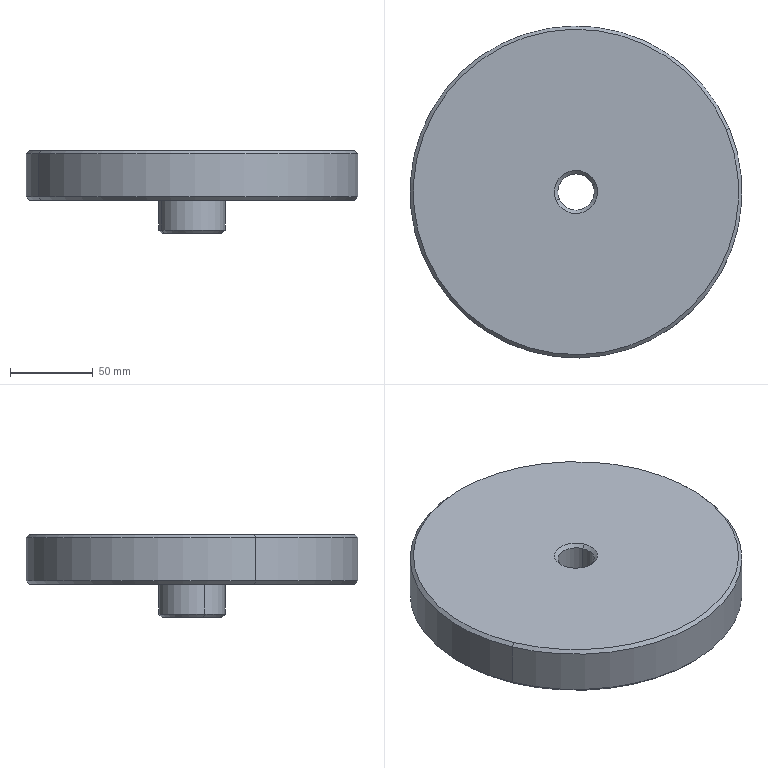Component | SolidWorks | Pinion-1 | 1 solid | 19 faces | box 200 x 200 x 50 mm | volume 945571 mm3 | cone 10 | cylinder 6 | plane 3 | commonest cylinder face diameters 40 x2 200 x2 22 x2 | material 45
build123d program:
from build123d import *

# Parameters (mm, degrees)
CHAMFER1_SIZE = 2


with BuildPart() as part:
    # Sketch1 → Revolve1 (revolve)
    with BuildSketch(Plane.XY, mode=Mode.PRIVATE) as revolve1_sk:
        Polygon((0, 11), (0, 100), (30, 100), (30, 20), (50, 20), (50, 11), align=None)
    revolve(revolve1_sk.sketch.rotate(Axis((0, 0, 0), (1, 0, 0)), 90), axis=Axis((0, 0, 0), (1, 0, 0)))

    # Chamfer1
    chamfer1_edges = [part.edges().sort_by_distance(p)[0] for p in [
        (50, 0, -11),
        (50, 0, -20),
        (30, 0, -100),
        (0, 0, -100),
        (0, 0, -11),
    ]]
    chamfer(chamfer1_edges, length=CHAMFER1_SIZE)


solid = part.part

# Placed as in the assembly
solid = solid.moved(Location((110.202, 126.699, 572.267), (0, 90, 0)))
STEP:
#1=CARTESIAN_POINT('',(7.903,6.466,22.53));
#2=VERTEX_POINT('',#1);
#3=CARTESIAN_POINT('',(0.7747,3.51,22.53));
#4=VERTEX_POINT('',#3);
#5=CARTESIAN_POINT('',(4.339,4.988,22.53));
#6=DIRECTION('',(0.,-0.,1.));
#7=DIRECTION('',(-0.9237,-0.383,0.));
#8=AXIS2_PLACEMENT_3D('',#5,#6,#7);
#9=CIRCLE('',#8,3.858);
#10=EDGE_CURVE('',#2,#4,#9,.T.);
#11=ORIENTED_EDGE('',*,*,#10,.F.);
#12=CARTESIAN_POINT('',(7.975,6.496,22.451));
#13=VERTEX_POINT('',#12);
#14=CARTESIAN_POINT('',(7.903,6.466,22.53));
#15=DIRECTION('',(0.6532,0.2709,-0.7071));
#16=VECTOR('',#15,39.37);
#17=LINE('',#14,#16);
#18=EDGE_CURVE('',#2,#13,#17,.T.);
#19=ORIENTED_EDGE('',*,*,#18,.T.);
#20=CARTESIAN_POINT('',(0.7019,3.48,22.451));
#21=VERTEX_POINT('',#20);
#22=CARTESIAN_POINT('',(4.339,4.988,22.451));
#23=DIRECTION('',(-0.,0.,-1.));
#24=DIRECTION('',(-0.9237,-0.383,0.));
#25=AXIS2_PLACEMENT_3D('',#22,#23,#24);
#26=CIRCLE('',#25,3.937);
#27=EDGE_CURVE('',#21,#13,#26,.T.);
#28=ORIENTED_EDGE('',*,*,#27,.F.);
#29=CARTESIAN_POINT('',(0.7747,3.51,22.53));
#30=DIRECTION('',(-0.6532,-0.2709,-0.7071));
#31=VECTOR('',#30,39.37);
#32=LINE('',#29,#31);
#33=EDGE_CURVE('',#4,#21,#32,.T.);
#34=ORIENTED_EDGE('',*,*,#33,.F.);
#35=EDGE_LOOP('',(#11,#19,#28,#34));
#36=FACE_OUTER_BOUND('',#35,.T.);
#37=CARTESIAN_POINT('',(4.339,4.988,22.53));
#38=DIRECTION('',(-0.,0.,-1.));
#39=DIRECTION('',(-0.9237,-0.383,0.));
#40=AXIS2_PLACEMENT_3D('',#37,#38,#39);
#41=CONICAL_SURFACE('',#40,3.858,0.7854);
#42=ADVANCED_FACE('',(#36),#41,.T.);
#43=CARTESIAN_POINT('',(0.7747,3.51,21.349));
#44=VERTEX_POINT('',#43);
#45=CARTESIAN_POINT('',(7.903,6.466,21.349));
#46=VERTEX_POINT('',#45);
#47=CARTESIAN_POINT('',(4.339,4.988,21.349));
#48=DIRECTION('',(-0.,0.,-1.));
#49=DIRECTION('',(0.9237,0.383,0.));
#50=AXIS2_PLACEMENT_3D('',#47,#48,#49);
#51=CIRCLE('',#50,3.858);
#52=EDGE_CURVE('',#44,#46,#51,.T.);
#53=ORIENTED_EDGE('',*,*,#52,.F.);
#54=CARTESIAN_POINT('',(0.7019,3.48,21.428));
#55=VERTEX_POINT('',#54);
#56=CARTESIAN_POINT('',(0.7019,3.48,21.428));
#57=DIRECTION('',(-0.6532,-0.2709,0.7071));
#58=VECTOR('',#57,39.37);
#59=LINE('',#56,#58);
#60=EDGE_CURVE('',#44,#55,#59,.T.);
#61=ORIENTED_EDGE('',*,*,#60,.T.);
#62=CARTESIAN_POINT('',(7.975,6.496,21.428));
#63=VERTEX_POINT('',#62);
#64=CARTESIAN_POINT('',(4.339,4.988,21.428));
#65=DIRECTION('',(0.,-0.,1.));
#66=DIRECTION('',(0.9237,0.383,0.));
#67=AXIS2_PLACEMENT_3D('',#64,#65,#66);
#68=CIRCLE('',#67,3.937);
#69=EDGE_CURVE('',#63,#55,#68,.T.);
#70=ORIENTED_EDGE('',*,*,#69,.F.);
#71=CARTESIAN_POINT('',(7.975,6.496,21.428));
#72=DIRECTION('',(0.6532,0.2709,0.7071));
#73=VECTOR('',#72,39.37);
#74=LINE('',#71,#73);
#75=EDGE_CURVE('',#46,#63,#74,.T.);
#76=ORIENTED_EDGE('',*,*,#75,.F.);
#77=EDGE_LOOP('',(#53,#61,#70,#76));
#78=FACE_OUTER_BOUND('',#77,.T.);
#79=CARTESIAN_POINT('',(4.339,4.988,21.428));
#80=DIRECTION('',(0.,-0.,1.));
#81=DIRECTION('',(0.9237,0.383,0.));
#82=AXIS2_PLACEMENT_3D('',#79,#80,#81);
#83=CONICAL_SURFACE('',#82,3.937,0.7854);
#84=ADVANCED_FACE('',(#78),#83,.T.);
#85=CARTESIAN_POINT('',(3.684,4.717,20.562));
#86=VERTEX_POINT('',#85);
#87=CARTESIAN_POINT('',(4.993,5.26,20.562));
#88=VERTEX_POINT('',#87);
#89=CARTESIAN_POINT('',(4.339,4.988,20.562));
#90=DIRECTION('',(-0.,0.,-1.));
#91=DIRECTION('',(0.9237,0.383,0.));
#92=AXIS2_PLACEMENT_3D('',#89,#90,#91);
#93=CIRCLE('',#92,0.7087);
#94=EDGE_CURVE('',#86,#88,#93,.T.);
#95=ORIENTED_EDGE('',*,*,#94,.F.);
#96=CARTESIAN_POINT('',(3.611,4.687,20.64));
#97=VERTEX_POINT('',#96);
#98=CARTESIAN_POINT('',(3.611,4.687,20.64));
#99=DIRECTION('',(-0.6532,-0.2709,0.7071));
#100=VECTOR('',#99,39.37);
#101=LINE('',#98,#100);
#102=EDGE_CURVE('',#86,#97,#101,.T.);
#103=ORIENTED_EDGE('',*,*,#102,.T.);
#104=CARTESIAN_POINT('',(5.066,5.29,20.64));
#105=VERTEX_POINT('',#104);
#106=CARTESIAN_POINT('',(4.339,4.988,20.64));
#107=DIRECTION('',(0.,-0.,1.));
#108=DIRECTION('',(0.9237,0.383,0.));
#109=AXIS2_PLACEMENT_3D('',#106,#107,#108);
#110=CIRCLE('',#109,0.7874);
#111=EDGE_CURVE('',#105,#97,#110,.T.);
#112=ORIENTED_EDGE('',*,*,#111,.F.);
#113=CARTESIAN_POINT('',(5.066,5.29,20.64));
#114=DIRECTION('',(0.6532,0.2709,0.7071));
#115=VECTOR('',#114,39.37);
#116=LINE('',#113,#115);
#117=EDGE_CURVE('',#88,#105,#116,.T.);
#118=ORIENTED_EDGE('',*,*,#117,.F.);
#119=EDGE_LOOP('',(#95,#103,#112,#118));
#120=FACE_OUTER_BOUND('',#119,.T.);
#121=CARTESIAN_POINT('',(4.339,4.988,20.64));
#122=DIRECTION('',(0.,-0.,1.));
#123=DIRECTION('',(0.9237,0.383,0.));
#124=AXIS2_PLACEMENT_3D('',#121,#122,#123);
#125=CONICAL_SURFACE('',#124,0.7874,0.7854);
#126=ADVANCED_FACE('',(#120),#125,.T.);
#127=CARTESIAN_POINT('',(4.739,5.154,20.64));
#128=VERTEX_POINT('',#127);
#129=CARTESIAN_POINT('',(3.939,4.822,20.64));
#130=VERTEX_POINT('',#129);
#131=CARTESIAN_POINT('',(4.339,4.988,20.64));
#132=DIRECTION('',(-0.,0.,-1.));
#133=DIRECTION('',(0.9237,0.383,0.));
#134=AXIS2_PLACEMENT_3D('',#131,#132,#133);
#135=CIRCLE('',#134,0.4331);
#136=EDGE_CURVE('',#128,#130,#135,.T.);
#137=ORIENTED_EDGE('',*,*,#136,.F.);
#138=CARTESIAN_POINT('',(4.811,5.184,20.562));
#139=VERTEX_POINT('',#138);
#140=CARTESIAN_POINT('',(4.811,5.184,20.562));
#141=DIRECTION('',(0.6532,0.2709,-0.7071));
#142=VECTOR('',#141,39.37);
#143=LINE('',#140,#142);
#144=EDGE_CURVE('',#128,#139,#143,.T.);
#145=ORIENTED_EDGE('',*,*,#144,.T.);
#146=CARTESIAN_POINT('',(3.866,4.792,20.562));
#147=VERTEX_POINT('',#146);
#148=CARTESIAN_POINT('',(4.339,4.988,20.562));
#149=DIRECTION('',(0.,-0.,1.));
#150=DIRECTION('',(0.9237,0.383,0.));
#151=AXIS2_PLACEMENT_3D('',#148,#149,#150);
#152=CIRCLE('',#151,0.5118);
#153=EDGE_CURVE('',#147,#139,#152,.T.);
#154=ORIENTED_EDGE('',*,*,#153,.F.);
#155=CARTESIAN_POINT('',(3.866,4.792,20.562));
#156=DIRECTION('',(-0.6532,-0.2709,-0.7071));
#157=VECTOR('',#156,39.37);
#158=LINE('',#155,#157);
#159=EDGE_CURVE('',#130,#147,#158,.T.);
#160=ORIENTED_EDGE('',*,*,#159,.F.);
#161=EDGE_LOOP('',(#137,#145,#154,#160));
#162=FACE_OUTER_BOUND('',#161,.T.);
#163=CARTESIAN_POINT('',(4.339,4.988,20.562));
#164=DIRECTION('',(-0.,0.,-1.));
#165=DIRECTION('',(-0.9237,-0.383,0.));
#166=AXIS2_PLACEMENT_3D('',#163,#164,#165);
#167=CONICAL_SURFACE('',#166,0.5118,0.7854);
#168=ADVANCED_FACE('',(#162),#167,.F.);
#169=CARTESIAN_POINT('',(3.939,4.822,22.451));
#170=VERTEX_POINT('',#169);
#171=CARTESIAN_POINT('',(4.739,5.154,22.451));
#172=VERTEX_POINT('',#171);
#173=CARTESIAN_POINT('',(4.339,4.988,22.451));
#174=DIRECTION('',(0.,-0.,1.));
#175=DIRECTION('',(-0.9237,-0.383,0.));
#176=AXIS2_PLACEMENT_3D('',#173,#174,#175);
#177=CIRCLE('',#176,0.4331);
#178=EDGE_CURVE('',#170,#172,#177,.T.);
#179=ORIENTED_EDGE('',*,*,#178,.F.);
#180=CARTESIAN_POINT('',(3.866,4.792,22.53));
#181=VERTEX_POINT('',#180);
#182=CARTESIAN_POINT('',(3.939,4.822,22.451));
#183=DIRECTION('',(-0.6532,-0.2709,0.7071));
#184=VECTOR('',#183,39.37);
#185=LINE('',#182,#184);
#186=EDGE_CURVE('',#170,#181,#185,.T.);
#187=ORIENTED_EDGE('',*,*,#186,.T.);
#188=CARTESIAN_POINT('',(4.811,5.184,22.53));
#189=VERTEX_POINT('',#188);
#190=CARTESIAN_POINT('',(4.339,4.988,22.53));
#191=DIRECTION('',(-0.,0.,-1.));
#192=DIRECTION('',(-0.9237,-0.383,0.));
#193=AXIS2_PLACEMENT_3D('',#190,#191,#192);
#194=CIRCLE('',#193,0.5118);
#195=EDGE_CURVE('',#189,#181,#194,.T.);
#196=ORIENTED_EDGE('',*,*,#195,.F.);
#197=CARTESIAN_POINT('',(4.739,5.154,22.451));
#198=DIRECTION('',(0.6532,0.2709,0.7071));
#199=VECTOR('',#198,39.37);
#200=LINE('',#197,#199);
#201=EDGE_CURVE('',#172,#189,#200,.T.);
#202=ORIENTED_EDGE('',*,*,#201,.F.);
#203=EDGE_LOOP('',(#179,#187,#196,#202));
#204=FACE_OUTER_BOUND('',#203,.T.);
#205=CARTESIAN_POINT('',(4.339,4.988,22.451));
#206=DIRECTION('',(0.,-0.,1.));
#207=DIRECTION('',(0.9237,0.383,0.));
#208=AXIS2_PLACEMENT_3D('',#205,#206,#207);
#209=CONICAL_SURFACE('',#208,0.4331,0.7854);
#210=ADVANCED_FACE('',(#204),#209,.F.);
#211=ORIENTED_EDGE('',*,*,#111,.T.);
#212=CARTESIAN_POINT('',(3.611,4.687,21.349));
#213=VERTEX_POINT('',#212);
#214=CARTESIAN_POINT('',(3.611,4.687,22.53));
#215=DIRECTION('',(0.,-0.,1.));
#216=VECTOR('',#215,39.37);
#217=LINE('',#214,#216);
#218=EDGE_CURVE('',#97,#213,#217,.T.);
#219=ORIENTED_EDGE('',*,*,#218,.T.);
#220=CARTESIAN_POINT('',(5.066,5.29,21.349));
#221=VERTEX_POINT('',#220);
#222=CARTESIAN_POINT('',(4.339,4.988,21.349));
#223=DIRECTION('',(0.,-0.,1.));
#224=DIRECTION('',(0.9237,0.383,0.));
#225=AXIS2_PLACEMENT_3D('',#222,#223,#224);
#226=CIRCLE('',#225,0.7874);
#227=EDGE_CURVE('',#221,#213,#226,.T.);
#228=ORIENTED_EDGE('',*,*,#227,.F.);
#229=CARTESIAN_POINT('',(5.066,5.29,22.53));
#230=DIRECTION('',(0.,-0.,1.));
#231=VECTOR('',#230,39.37);
#232=LINE('',#229,#231);
#233=EDGE_CURVE('',#105,#221,#232,.T.);
#234=ORIENTED_EDGE('',*,*,#233,.F.);
#235=EDGE_LOOP('',(#211,#219,#228,#234));
#236=FACE_OUTER_BOUND('',#235,.T.);
#237=CARTESIAN_POINT('',(4.339,4.988,22.53));
#238=DIRECTION('',(0.,-0.,1.));
#239=DIRECTION('',(0.9237,0.383,0.));
#240=AXIS2_PLACEMENT_3D('',#237,#238,#239);
#241=CYLINDRICAL_SURFACE('',#240,0.7874);
#242=ADVANCED_FACE('',(#236),#241,.T.);
#243=ORIENTED_EDGE('',*,*,#69,.T.);
#244=CARTESIAN_POINT('',(0.7019,3.48,22.53));
#245=DIRECTION('',(0.,-0.,1.));
#246=VECTOR('',#245,39.37);
#247=LINE('',#244,#246);
#248=EDGE_CURVE('',#55,#21,#247,.T.);
#249=ORIENTED_EDGE('',*,*,#248,.T.);
#250=ORIENTED_EDGE('',*,*,#27,.T.);
#251=CARTESIAN_POINT('',(7.975,6.496,22.53));
#252=DIRECTION('',(0.,-0.,1.));
#253=VECTOR('',#252,39.37);
#254=LINE('',#251,#253);
#255=EDGE_CURVE('',#63,#13,#254,.T.);
#256=ORIENTED_EDGE('',*,*,#255,.F.);
#257=EDGE_LOOP('',(#243,#249,#250,#256));
#258=FACE_OUTER_BOUND('',#257,.T.);
#259=CARTESIAN_POINT('',(4.339,4.988,22.53));
#260=DIRECTION('',(0.,-0.,1.));
#261=DIRECTION('',(0.9237,0.383,0.));
#262=AXIS2_PLACEMENT_3D('',#259,#260,#261);
#263=CYLINDRICAL_SURFACE('',#262,3.937);
#264=ADVANCED_FACE('',(#258),#263,.T.);
#265=ORIENTED_EDGE('',*,*,#136,.T.);
#266=CARTESIAN_POINT('',(3.939,4.822,22.53));
#267=DIRECTION('',(0.,-0.,1.));
#268=VECTOR('',#267,39.37);
#269=LINE('',#266,#268);
#270=EDGE_CURVE('',#130,#170,#269,.T.);
#271=ORIENTED_EDGE('',*,*,#270,.T.);
#272=ORIENTED_EDGE('',*,*,#178,.T.);
#273=CARTESIAN_POINT('',(4.739,5.154,22.53));
#274=DIRECTION('',(0.,-0.,1.));
#275=VECTOR('',#274,39.37);
#276=LINE('',#273,#275);
#277=EDGE_CURVE('',#128,#172,#276,.T.);
#278=ORIENTED_EDGE('',*,*,#277,.F.);
#279=EDGE_LOOP('',(#265,#271,#272,#278));
#280=FACE_OUTER_BOUND('',#279,.T.);
#281=CARTESIAN_POINT('',(4.339,4.988,22.53));
#282=DIRECTION('',(0.,-0.,1.));
#283=DIRECTION('',(0.9237,0.383,0.));
#284=AXIS2_PLACEMENT_3D('',#281,#282,#283);
#285=CYLINDRICAL_SURFACE('',#284,0.4331);
#286=ADVANCED_FACE('',(#280),#285,.F.);
#287=ORIENTED_EDGE('',*,*,#270,.F.);
#288=CARTESIAN_POINT('',(4.339,4.988,20.64));
#289=DIRECTION('',(-0.,0.,-1.));
#290=DIRECTION('',(0.9237,0.383,0.));
#291=AXIS2_PLACEMENT_3D('',#288,#289,#290);
#292=CIRCLE('',#291,0.4331);
#293=EDGE_CURVE('',#130,#128,#292,.T.);
#294=ORIENTED_EDGE('',*,*,#293,.T.);
#295=ORIENTED_EDGE('',*,*,#277,.T.);
#296=CARTESIAN_POINT('',(4.339,4.988,22.451));
#297=DIRECTION('',(0.,-0.,1.));
#298=DIRECTION('',(-0.9237,-0.383,0.));
#299=AXIS2_PLACEMENT_3D('',#296,#297,#298);
#300=CIRCLE('',#299,0.4331);
#301=EDGE_CURVE('',#172,#170,#300,.T.);
#302=ORIENTED_EDGE('',*,*,#301,.T.);
#303=EDGE_LOOP('',(#287,#294,#295,#302));
#304=FACE_OUTER_BOUND('',#303,.T.);
#305=CARTESIAN_POINT('',(4.339,4.988,22.53));
#306=DIRECTION('',(0.,-0.,1.));
#307=DIRECTION('',(0.9237,0.383,0.));
#308=AXIS2_PLACEMENT_3D('',#305,#306,#307);
#309=CYLINDRICAL_SURFACE('',#308,0.4331);
#310=ADVANCED_FACE('',(#304),#309,.F.);
#311=ORIENTED_EDGE('',*,*,#195,.T.);
#312=CARTESIAN_POINT('',(4.339,4.988,22.53));
#313=DIRECTION('',(-0.,0.,-1.));
#314=DIRECTION('',(-0.9237,-0.383,0.));
#315=AXIS2_PLACEMENT_3D('',#312,#313,#314);
#316=CIRCLE('',#315,0.5118);
#317=EDGE_CURVE('',#181,#189,#316,.T.);
#318=ORIENTED_EDGE('',*,*,#317,.T.);
#319=EDGE_LOOP('',(#311,#318));
#320=FACE_BOUND('',#319,.T.);
#321=CARTESIAN_POINT('',(4.339,4.988,22.53));
#322=DIRECTION('',(0.,-0.,1.));
#323=DIRECTION('',(-0.9237,-0.383,0.));
#324=AXIS2_PLACEMENT_3D('',#321,#322,#323);
#325=CIRCLE('',#324,3.858);
#326=EDGE_CURVE('',#4,#2,#325,.T.);
#327=ORIENTED_EDGE('',*,*,#326,.T.);
#328=ORIENTED_EDGE('',*,*,#10,.T.);
#329=EDGE_LOOP('',(#327,#328));
#330=FACE_OUTER_BOUND('',#329,.T.);
#331=CARTESIAN_POINT('',(4.173,5.388,22.53));
#332=DIRECTION('',(-0.,0.,-1.));
#333=DIRECTION('',(-0.9237,-0.383,0.));
#334=AXIS2_PLACEMENT_3D('',#331,#332,#333);
#335=PLANE('',#334);
#336=ADVANCED_FACE('',(#320,#330),#335,.F.);
#337=ORIENTED_EDGE('',*,*,#248,.F.);
#338=CARTESIAN_POINT('',(4.339,4.988,21.428));
#339=DIRECTION('',(0.,-0.,1.));
#340=DIRECTION('',(0.9237,0.383,0.));
#341=AXIS2_PLACEMENT_3D('',#338,#339,#340);
#342=CIRCLE('',#341,3.937);
#343=EDGE_CURVE('',#55,#63,#342,.T.);
#344=ORIENTED_EDGE('',*,*,#343,.T.);
#345=ORIENTED_EDGE('',*,*,#255,.T.);
#346=CARTESIAN_POINT('',(4.339,4.988,22.451));
#347=DIRECTION('',(-0.,0.,-1.));
#348=DIRECTION('',(-0.9237,-0.383,0.));
#349=AXIS2_PLACEMENT_3D('',#346,#347,#348);
#350=CIRCLE('',#349,3.937);
#351=EDGE_CURVE('',#13,#21,#350,.T.);
#352=ORIENTED_EDGE('',*,*,#351,.T.);
#353=EDGE_LOOP('',(#337,#344,#345,#352));
#354=FACE_OUTER_BOUND('',#353,.T.);
#355=CARTESIAN_POINT('',(4.339,4.988,22.53));
#356=DIRECTION('',(0.,-0.,1.));
#357=DIRECTION('',(0.9237,0.383,0.));
#358=AXIS2_PLACEMENT_3D('',#355,#356,#357);
#359=CYLINDRICAL_SURFACE('',#358,3.937);
#360=ADVANCED_FACE('',(#354),#359,.T.);
#361=CARTESIAN_POINT('',(4.339,4.988,21.349));
#362=DIRECTION('',(-0.,0.,-1.));
#363=DIRECTION('',(0.9237,0.383,0.));
#364=AXIS2_PLACEMENT_3D('',#361,#362,#363);
#365=CIRCLE('',#364,3.858);
#366=EDGE_CURVE('',#46,#44,#365,.T.);
#367=ORIENTED_EDGE('',*,*,#366,.T.);
#368=ORIENTED_EDGE('',*,*,#52,.T.);
#369=EDGE_LOOP('',(#367,#368));
#370=FACE_OUTER_BOUND('',#369,.T.);
#371=ORIENTED_EDGE('',*,*,#227,.T.);
#372=CARTESIAN_POINT('',(4.339,4.988,21.349));
#373=DIRECTION('',(0.,-0.,1.));
#374=DIRECTION('',(0.9237,0.383,0.));
#375=AXIS2_PLACEMENT_3D('',#372,#373,#374);
#376=CIRCLE('',#375,0.7874);
#377=EDGE_CURVE('',#213,#221,#376,.T.);
#378=ORIENTED_EDGE('',*,*,#377,.T.);
#379=EDGE_LOOP('',(#371,#378));
#380=FACE_BOUND('',#379,.T.);
#381=CARTESIAN_POINT('',(2.831,8.625,21.349));
#382=DIRECTION('',(0.,-0.,1.));
#383=DIRECTION('',(0.9237,0.383,-0.));
#384=AXIS2_PLACEMENT_3D('',#381,#382,#383);
#385=PLANE('',#384);
#386=ADVANCED_FACE('',(#370,#380),#385,.F.);
#387=ORIENTED_EDGE('',*,*,#218,.F.);
#388=CARTESIAN_POINT('',(4.339,4.988,20.64));
#389=DIRECTION('',(0.,-0.,1.));
#390=DIRECTION('',(0.9237,0.383,0.));
#391=AXIS2_PLACEMENT_3D('',#388,#389,#390);
#392=CIRCLE('',#391,0.7874);
#393=EDGE_CURVE('',#97,#105,#392,.T.);
#394=ORIENTED_EDGE('',*,*,#393,.T.);
#395=ORIENTED_EDGE('',*,*,#233,.T.);
#396=ORIENTED_EDGE('',*,*,#377,.F.);
#397=EDGE_LOOP('',(#387,#394,#395,#396));
#398=FACE_OUTER_BOUND('',#397,.T.);
#399=CARTESIAN_POINT('',(4.339,4.988,22.53));
#400=DIRECTION('',(0.,-0.,1.));
#401=DIRECTION('',(0.9237,0.383,0.));
#402=AXIS2_PLACEMENT_3D('',#399,#400,#401);
#403=CYLINDRICAL_SURFACE('',#402,0.7874);
#404=ADVANCED_FACE('',(#398),#403,.T.);
#405=ORIENTED_EDGE('',*,*,#153,.T.);
#406=CARTESIAN_POINT('',(4.339,4.988,20.562));
#407=DIRECTION('',(0.,-0.,1.));
#408=DIRECTION('',(0.9237,0.383,0.));
#409=AXIS2_PLACEMENT_3D('',#406,#407,#408);
#410=CIRCLE('',#409,0.5118);
#411=EDGE_CURVE('',#139,#147,#410,.T.);
#412=ORIENTED_EDGE('',*,*,#411,.T.);
#413=EDGE_LOOP('',(#405,#412));
#414=FACE_BOUND('',#413,.T.);
#415=CARTESIAN_POINT('',(4.339,4.988,20.562));
#416=DIRECTION('',(-0.,0.,-1.));
#417=DIRECTION('',(0.9237,0.383,0.));
#418=AXIS2_PLACEMENT_3D('',#415,#416,#417);
#419=CIRCLE('',#418,0.7087);
#420=EDGE_CURVE('',#88,#86,#419,.T.);
#421=ORIENTED_EDGE('',*,*,#420,.T.);
#422=ORIENTED_EDGE('',*,*,#94,.T.);
#423=EDGE_LOOP('',(#421,#422));
#424=FACE_OUTER_BOUND('',#423,.T.);
#425=CARTESIAN_POINT('',(4.037,5.716,20.562));
#426=DIRECTION('',(0.,-0.,1.));
#427=DIRECTION('',(0.9237,0.383,-0.));
#428=AXIS2_PLACEMENT_3D('',#425,#426,#427);
#429=PLANE('',#428);
#430=ADVANCED_FACE('',(#414,#424),#429,.F.);
#431=ORIENTED_EDGE('',*,*,#186,.F.);
#432=ORIENTED_EDGE('',*,*,#301,.F.);
#433=ORIENTED_EDGE('',*,*,#201,.T.);
#434=ORIENTED_EDGE('',*,*,#317,.F.);
#435=EDGE_LOOP('',(#431,#432,#433,#434));
#436=FACE_OUTER_BOUND('',#435,.T.);
#437=CARTESIAN_POINT('',(4.339,4.988,22.451));
#438=DIRECTION('',(0.,-0.,1.));
#439=DIRECTION('',(0.9237,0.383,0.));
#440=AXIS2_PLACEMENT_3D('',#437,#438,#439);
#441=CONICAL_SURFACE('',#440,0.4331,0.7854);
#442=ADVANCED_FACE('',(#436),#441,.F.);
#443=ORIENTED_EDGE('',*,*,#144,.F.);
#444=ORIENTED_EDGE('',*,*,#293,.F.);
#445=ORIENTED_EDGE('',*,*,#159,.T.);
#446=ORIENTED_EDGE('',*,*,#411,.F.);
#447=EDGE_LOOP('',(#443,#444,#445,#446));
#448=FACE_OUTER_BOUND('',#447,.T.);
#449=CARTESIAN_POINT('',(4.339,4.988,20.562));
#450=DIRECTION('',(-0.,0.,-1.));
#451=DIRECTION('',(-0.9237,-0.383,0.));
#452=AXIS2_PLACEMENT_3D('',#449,#450,#451);
#453=CONICAL_SURFACE('',#452,0.5118,0.7854);
#454=ADVANCED_FACE('',(#448),#453,.F.);
#455=ORIENTED_EDGE('',*,*,#102,.F.);
#456=ORIENTED_EDGE('',*,*,#420,.F.);
#457=ORIENTED_EDGE('',*,*,#117,.T.);
#458=ORIENTED_EDGE('',*,*,#393,.F.);
#459=EDGE_LOOP('',(#455,#456,#457,#458));
#460=FACE_OUTER_BOUND('',#459,.T.);
#461=CARTESIAN_POINT('',(4.339,4.988,20.64));
#462=DIRECTION('',(0.,-0.,1.));
#463=DIRECTION('',(0.9237,0.383,0.));
#464=AXIS2_PLACEMENT_3D('',#461,#462,#463);
#465=CONICAL_SURFACE('',#464,0.7874,0.7854);
#466=ADVANCED_FACE('',(#460),#465,.T.);
#467=ORIENTED_EDGE('',*,*,#60,.F.);
#468=ORIENTED_EDGE('',*,*,#366,.F.);
#469=ORIENTED_EDGE('',*,*,#75,.T.);
#470=ORIENTED_EDGE('',*,*,#343,.F.);
#471=EDGE_LOOP('',(#467,#468,#469,#470));
#472=FACE_OUTER_BOUND('',#471,.T.);
#473=CARTESIAN_POINT('',(4.339,4.988,21.428));
#474=DIRECTION('',(0.,-0.,1.));
#475=DIRECTION('',(0.9237,0.383,0.));
#476=AXIS2_PLACEMENT_3D('',#473,#474,#475);
#477=CONICAL_SURFACE('',#476,3.937,0.7854);
#478=ADVANCED_FACE('',(#472),#477,.T.);
#479=ORIENTED_EDGE('',*,*,#18,.F.);
#480=ORIENTED_EDGE('',*,*,#326,.F.);
#481=ORIENTED_EDGE('',*,*,#33,.T.);
#482=ORIENTED_EDGE('',*,*,#351,.F.);
#483=EDGE_LOOP('',(#479,#480,#481,#482));
#484=FACE_OUTER_BOUND('',#483,.T.);
#485=CARTESIAN_POINT('',(4.339,4.988,22.53));
#486=DIRECTION('',(-0.,0.,-1.));
#487=DIRECTION('',(-0.9237,-0.383,0.));
#488=AXIS2_PLACEMENT_3D('',#485,#486,#487);
#489=CONICAL_SURFACE('',#488,3.858,0.7854);
#490=ADVANCED_FACE('',(#484),#489,.T.);
#491=CLOSED_SHELL('',(#42,#84,#126,#168,#210,#242,#264,#286,#310,#336,#360,#386,#404,#430,#442,#454,#466,#478,#490));
#492=MANIFOLD_SOLID_BREP('',#491);
#493=CARTESIAN_POINT('',(0.,0.,0.));
#494=DIRECTION('',(0.,0.,1.));
#495=DIRECTION('',(1.,0.,0.));
#496=AXIS2_PLACEMENT_3D('',#493,#494,#495);
#497=(LENGTH_UNIT()NAMED_UNIT(*)SI_UNIT($,.METRE.));
#498=LENGTH_MEASURE_WITH_UNIT(LENGTH_MEASURE(0.0254),#497);
#499=DIMENSIONAL_EXPONENTS(1.,0.,0.,0.,0.,0.,0.);
#500=(CONVERSION_BASED_UNIT('',#498)LENGTH_UNIT()NAMED_UNIT(#499));
#501=UNCERTAINTY_MEASURE_WITH_UNIT(LENGTH_MEASURE(0.00001),#500,'','');
#502=(NAMED_UNIT(*)PLANE_ANGLE_UNIT()SI_UNIT($,.RADIAN.));
#503=(NAMED_UNIT(*)SI_UNIT($,.STERADIAN.)SOLID_ANGLE_UNIT());
#504=(GEOMETRIC_REPRESENTATION_CONTEXT(3)GLOBAL_UNCERTAINTY_ASSIGNED_CONTEXT((#501))GLOBAL_UNIT_ASSIGNED_CONTEXT((#500,#502,#503))REPRESENTATION_CONTEXT('',''));
#505=ADVANCED_BREP_SHAPE_REPRESENTATION('',(#492,#496),#504);
#506=COLOUR_RGB('',0.7922,0.8196,0.9333);
#507=FILL_AREA_STYLE_COLOUR('',#506);
#508=FILL_AREA_STYLE('',(#507));
#509=SURFACE_STYLE_FILL_AREA(#508);
#510=SURFACE_SIDE_STYLE('',(#509));
#511=SURFACE_STYLE_USAGE(.BOTH.,#510);
#512=PRESENTATION_STYLE_ASSIGNMENT((#511));
#513=STYLED_ITEM('',(#512),#492);
#514=(LENGTH_UNIT()NAMED_UNIT(*)SI_UNIT($,.METRE.));
#515=LENGTH_MEASURE_WITH_UNIT(LENGTH_MEASURE(0.0254),#514);
#516=DIMENSIONAL_EXPONENTS(1.,0.,0.,0.,0.,0.,0.);
#517=(CONVERSION_BASED_UNIT('',#515)LENGTH_UNIT()NAMED_UNIT(#516));
#518=UNCERTAINTY_MEASURE_WITH_UNIT(LENGTH_MEASURE(0.00001),#517,'','');
#519=(NAMED_UNIT(*)PLANE_ANGLE_UNIT()SI_UNIT($,.RADIAN.));
#520=(NAMED_UNIT(*)SI_UNIT($,.STERADIAN.)SOLID_ANGLE_UNIT());
#521=(GEOMETRIC_REPRESENTATION_CONTEXT(3)GLOBAL_UNCERTAINTY_ASSIGNED_CONTEXT((#518))GLOBAL_UNIT_ASSIGNED_CONTEXT((#517,#519,#520))REPRESENTATION_CONTEXT('',''));
#522=MECHANICAL_DESIGN_GEOMETRIC_PRESENTATION_REPRESENTATION('',(#513),#521);
#523=PRESENTATION_LAYER_ASSIGNMENT('','',(#513));